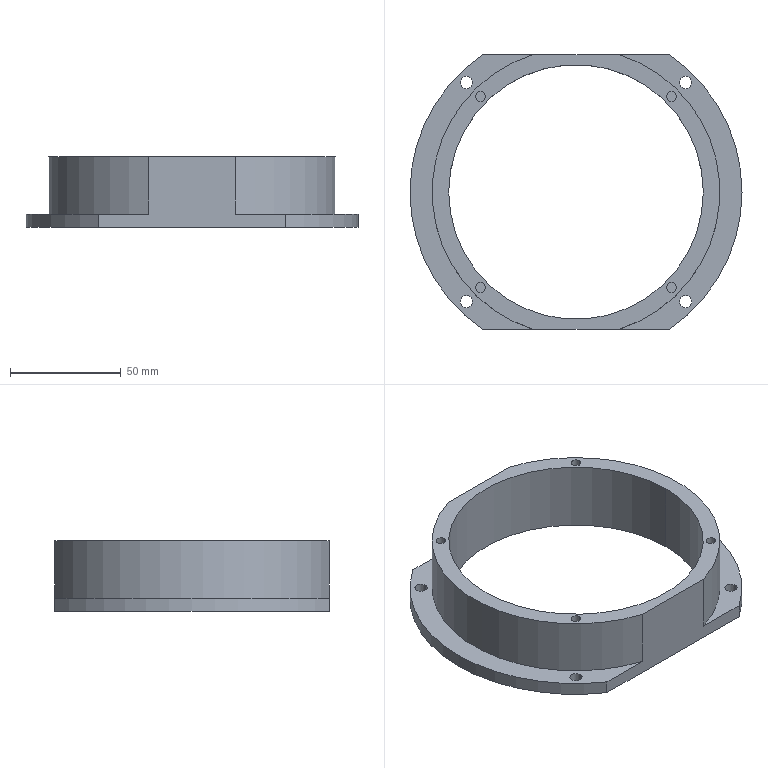CAM job | Mastercam | mm | 3 operations | part box 150 x 124 x 32
1. Contour (Ramp) | 13 - 16 平铣刀
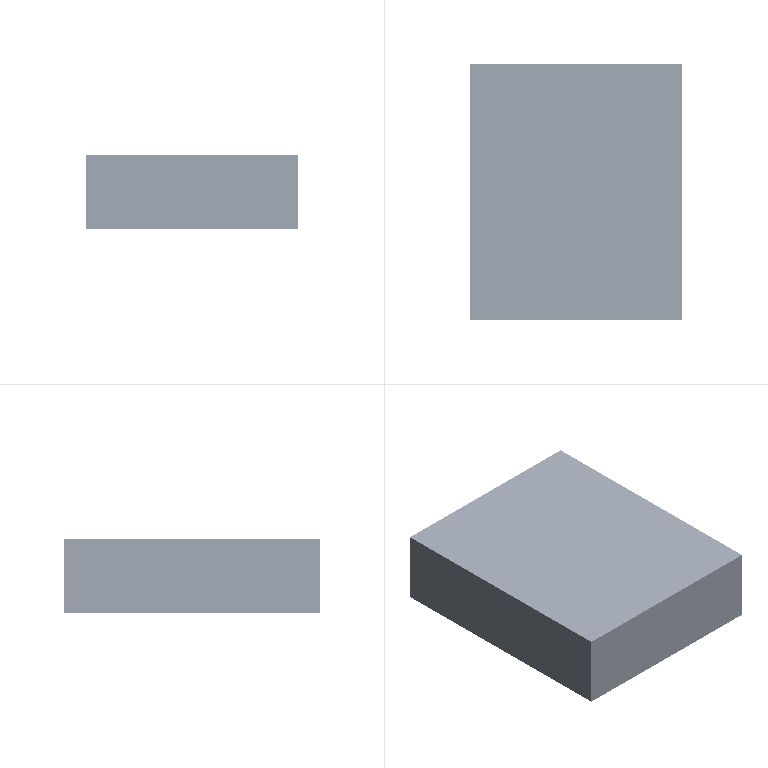2. Contour (2D) | 10 - 10 平铣刀
3. Drill/Counterbore | 7 - 6 倒角刀